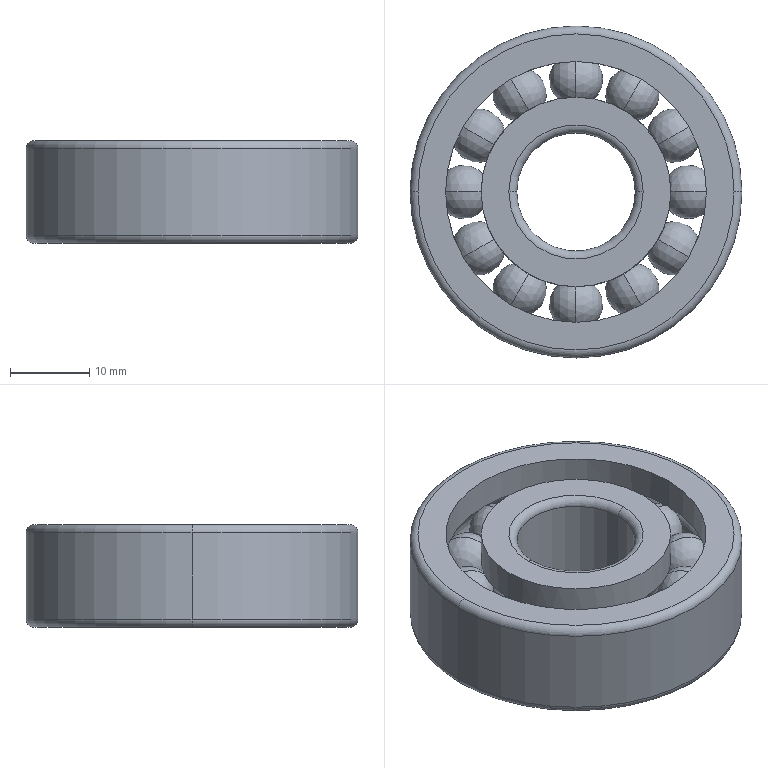Component | SolidWorks | Bearing-1 | 1 solid | 84 faces | box 42 x 42 x 13 mm | volume 11639 mm3 | torus 44 | sphere 24 | cylinder 12 | plane 4 | commonest cylinder face diameters 33 x4 24 x4 42 x2 15 x2
build123d program:
from build123d import *

# Parameters (mm, degrees)
CIRCULAR_PATTERN1_COUNT = 12
FILLET1_R               = 1


with BuildPart() as part:
    # Sketch1 → Revolve1 (revolve)
    with BuildSketch(Plane.XY):
        with BuildLine():
            Line((-3.375, 14.25), (3.375, 14.25))
            ThreePointArc((3.375, 14.25), (0, 17.625), (-3.375, 14.25))
        make_face()
    revolve1 = revolve(axis=Axis((-4.597, 14.25, 0), (1, 0, 0)))

    # Sketch2 → Revolve2 (revolve)
    with BuildSketch(Plane.XY, mode=Mode.PRIVATE) as revolve2_sk:
        with BuildLine():
            Line((-6.5, 12), (-6.5, 7.5))
            Line((-6.5, 7.5), (6.5, 7.5))
            Line((6.5, 7.5), (6.5, 12))
            Line((6.5, 12), (2.502, 12))
            ThreePointArc((2.502, 12), (0, 10.885), (-2.502, 12))
            Line((-2.502, 12), (-6.5, 12))
        make_face()
    revolve(revolve2_sk.sketch.rotate(Axis((-6.971, 0, 0), (1, 0, 0)), 90), axis=Axis((-6.971, 0, 0), (1, 0, 0)))

    # Sketch3 → Revolve3 (revolve)
    with BuildSketch(Plane.XY, mode=Mode.PRIVATE) as revolve3_sk:
        with BuildLine():
            Line((-6.5, 21), (6.5, 21))
            Line((6.5, 21), (6.5, 16.5))
            Line((6.5, 16.5), (2.502, 16.5))
            ThreePointArc((2.502, 16.5), (0, 17.615), (-2.502, 16.5))
            Line((-2.502, 16.5), (-6.5, 16.5))
            Line((-6.5, 16.5), (-6.5, 21))
        make_face()
    revolve(revolve3_sk.sketch.rotate(Axis((-8.711, 0, 0), (1, 0, 0)), 90), axis=Axis((-8.711, 0, 0), (1, 0, 0)))

    # Circular-Pattern1: Revolve1 ×12 about axis
    circular_pattern1_axis = Axis((0, 0, 0), (1, 0, 0))
    for i in range(1, CIRCULAR_PATTERN1_COUNT):
        add(revolve1.rotate(circular_pattern1_axis, i * 360 / CIRCULAR_PATTERN1_COUNT))

    # Fillet1
    fillet1_edges = [part.edges().sort_by_distance(p)[0] for p in [
        (-6.5, 0, -21),
        (6.5, 0, -21),
        (-6.5, 0, -7.5),
        (6.5, 0, -7.5),
    ]]
    fillet(fillet1_edges, radius=FILLET1_R)


solid = part.part

# Placed as in the assembly
solid = solid.moved(Location((113.982, -187.1, 35.962), (0, 90, 0)))